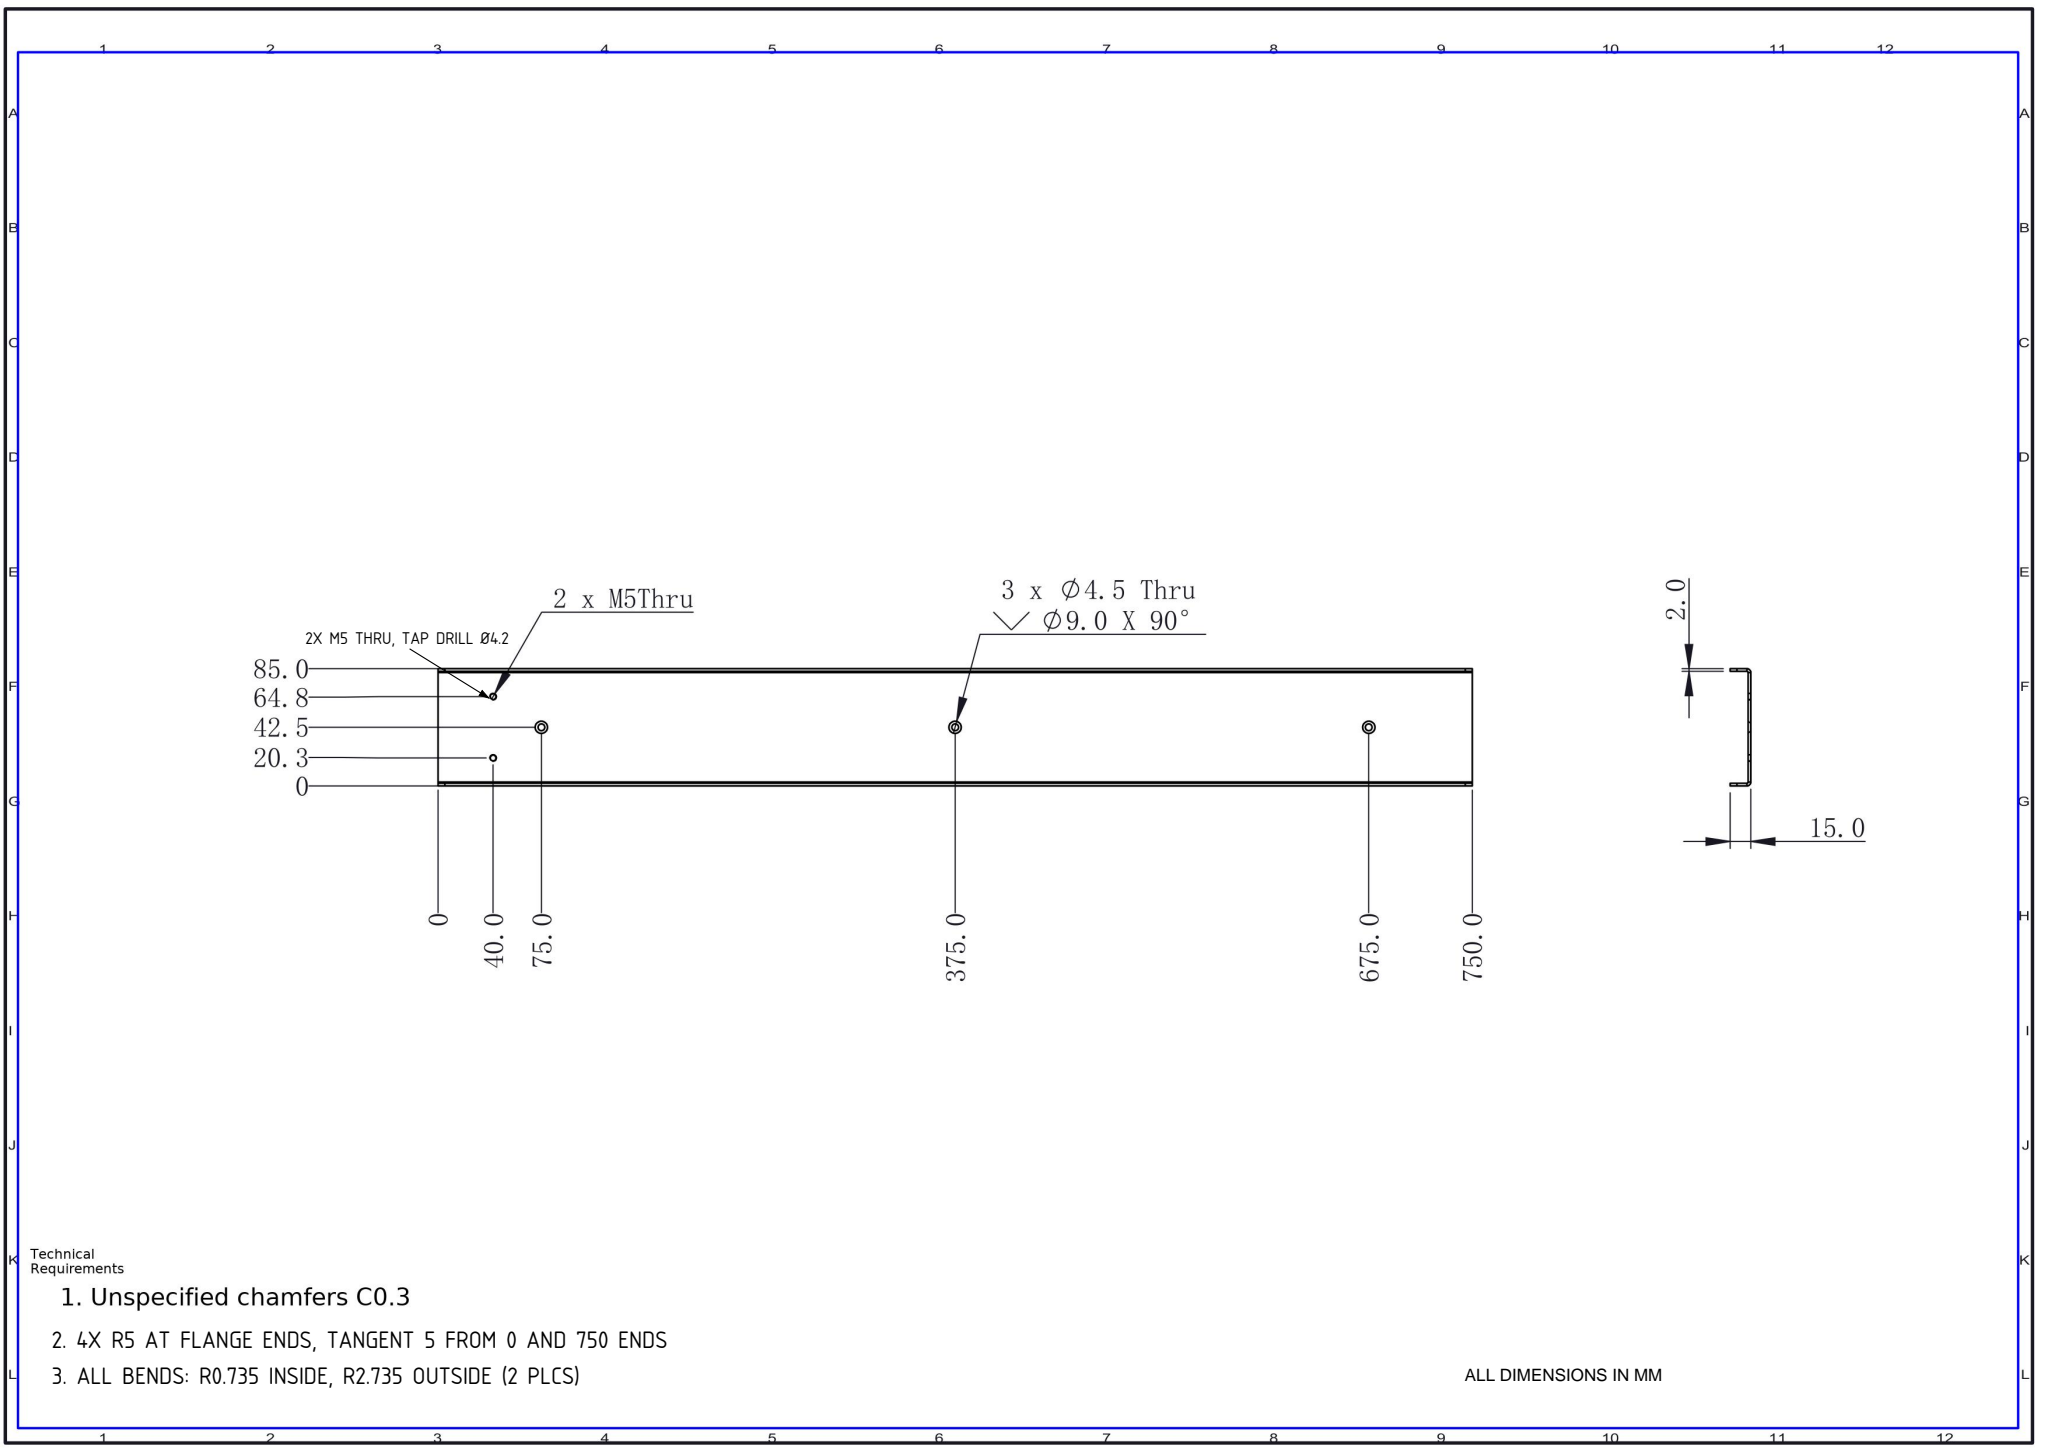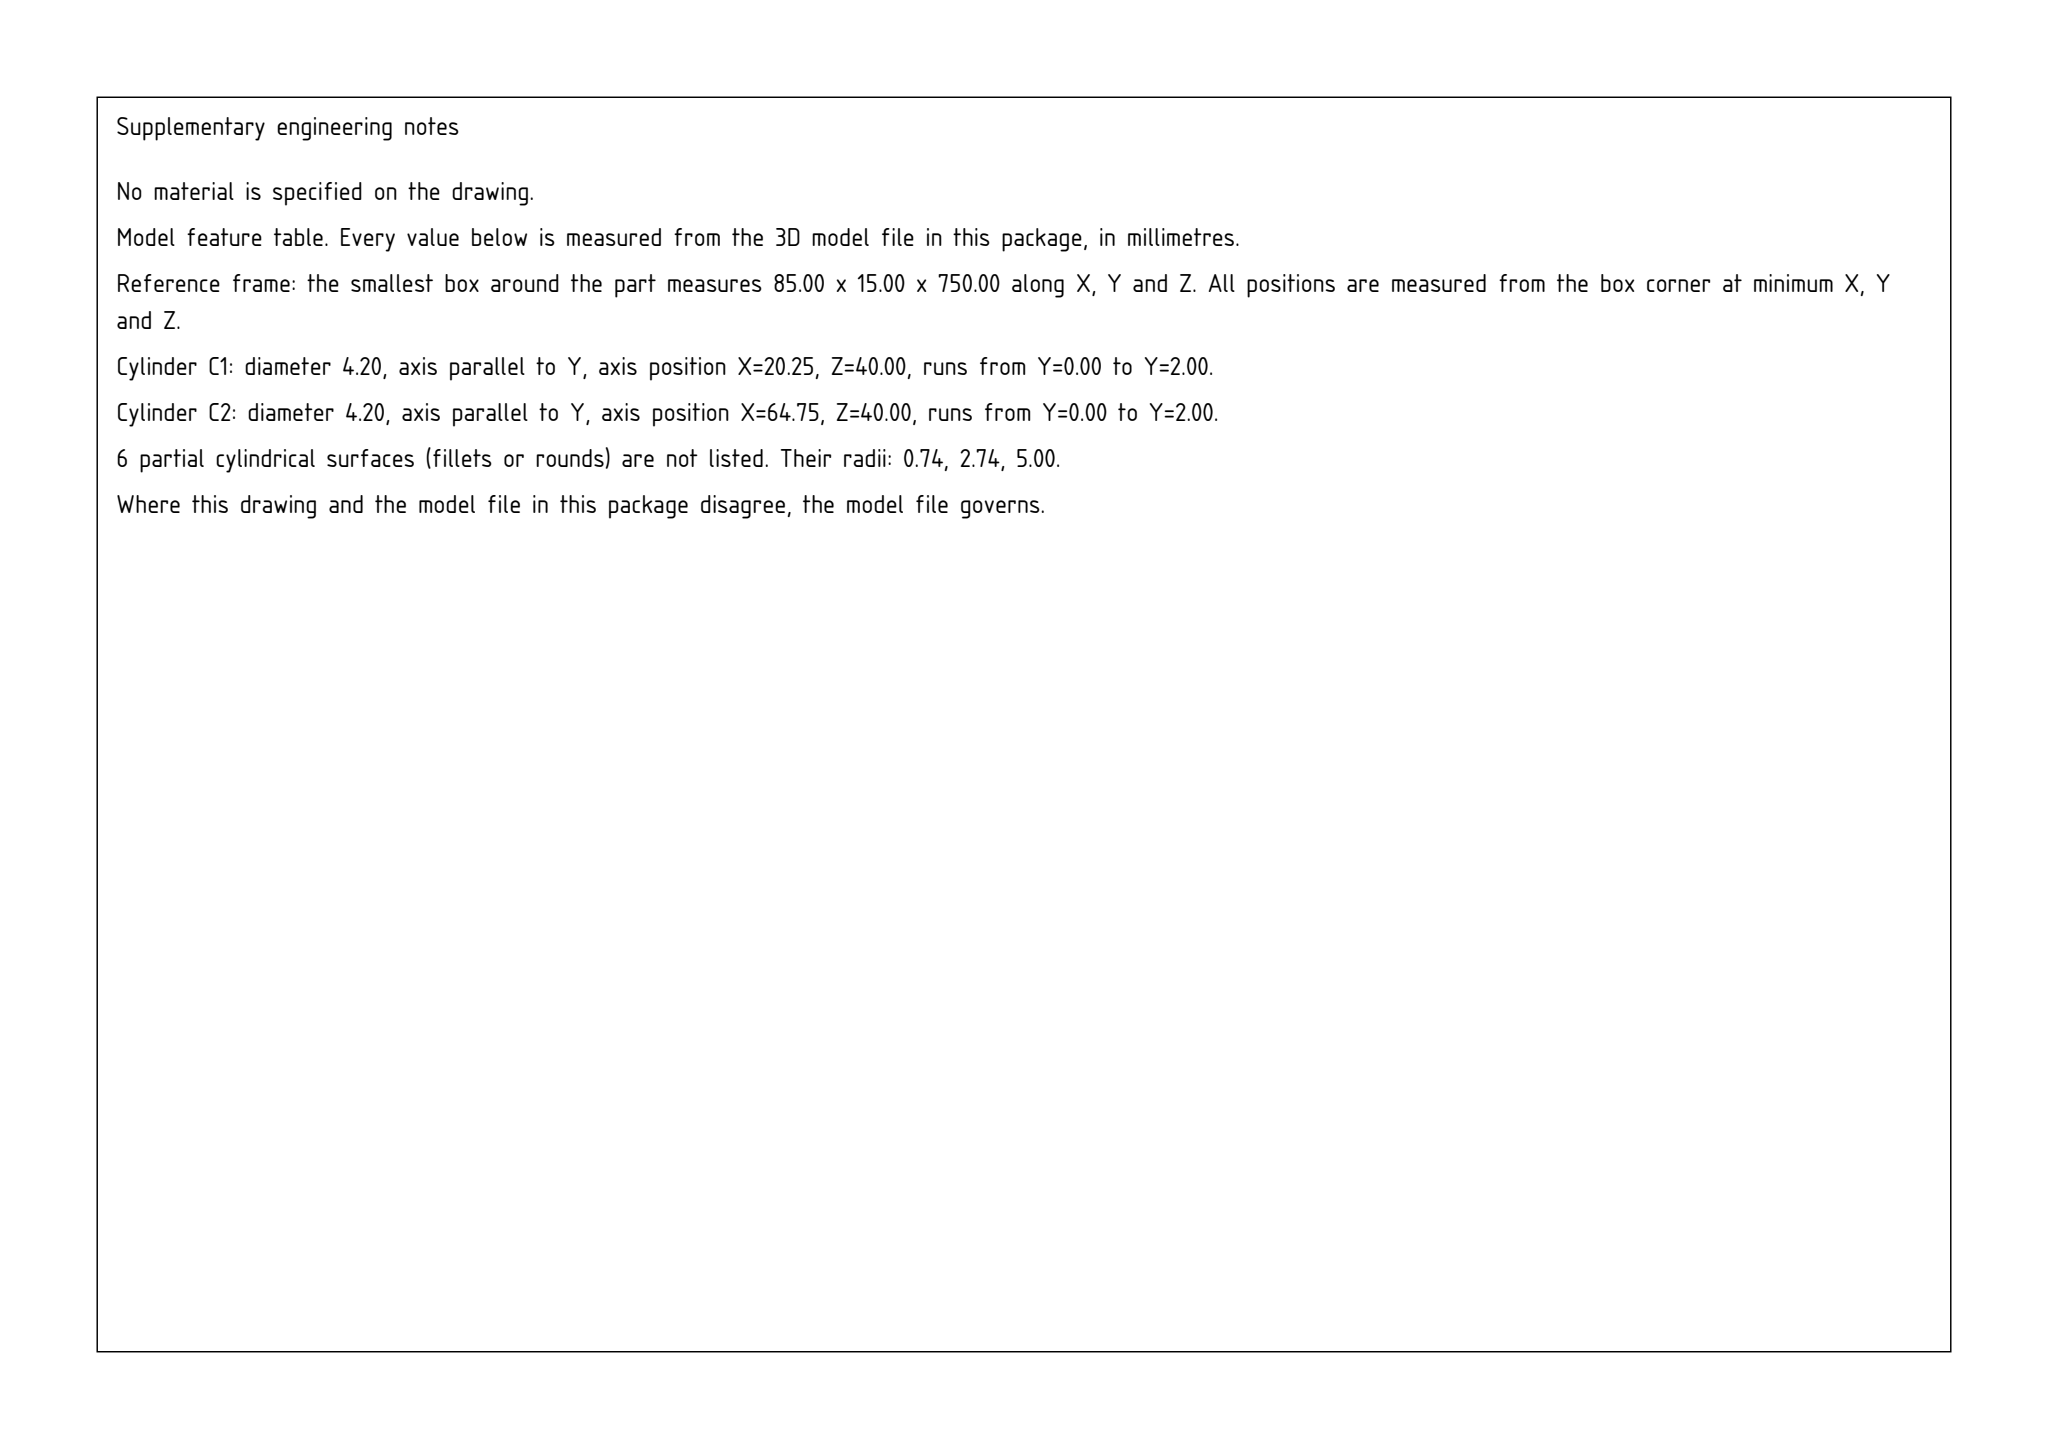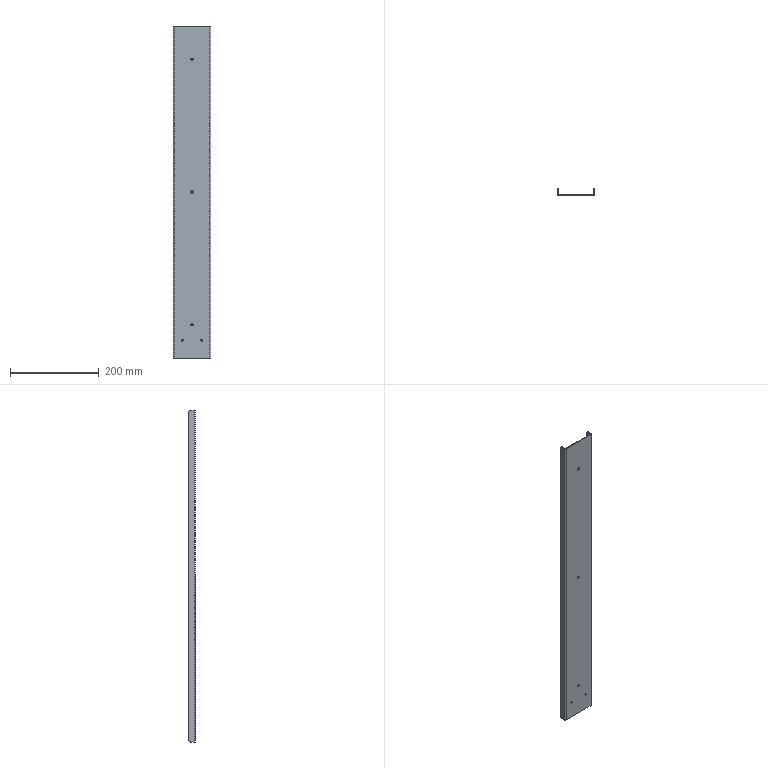Part | SolidWorks | mm | material SUS304 | 1 solid | 36 faces | box 85 x 15 x 750 mm | volume 163931 mm3 | plane 18 | cylinder 12 | cone 6 | commonest cylinder face diameters 4.2 x4 10 x4 5.473 x2 1.473 x2
Drawing notes:
4X R5 AT FLANGE ENDS, TANGENT 5 FROM 0 AND 750 ENDS | from the solid: convex arcs dia 10.0 (R5), axis x at y=10.0, z=5.0 and z=745.0, spanning x 0-2 and 83-85 (both flanges), 90 deg each
ALL BENDS: R0.735 INSIDE, R2.735 OUTSIDE (2 PLCS) | from the solid: Concave arc dia 1.47 (R0.735) at x=2.7,y=2.7 & x=82.3,y=2.7; convex arc dia 5.47 (R2.735) same axes, z 0-750
2 X M5 THRU (TAP DRILL Ø4.2 THRU 2.0 WALL) | from the solid: Two hole/bore Ø4.2, axis y, at (x20.3,z40) and (x64.8,z40), from y=0 to y=2.0